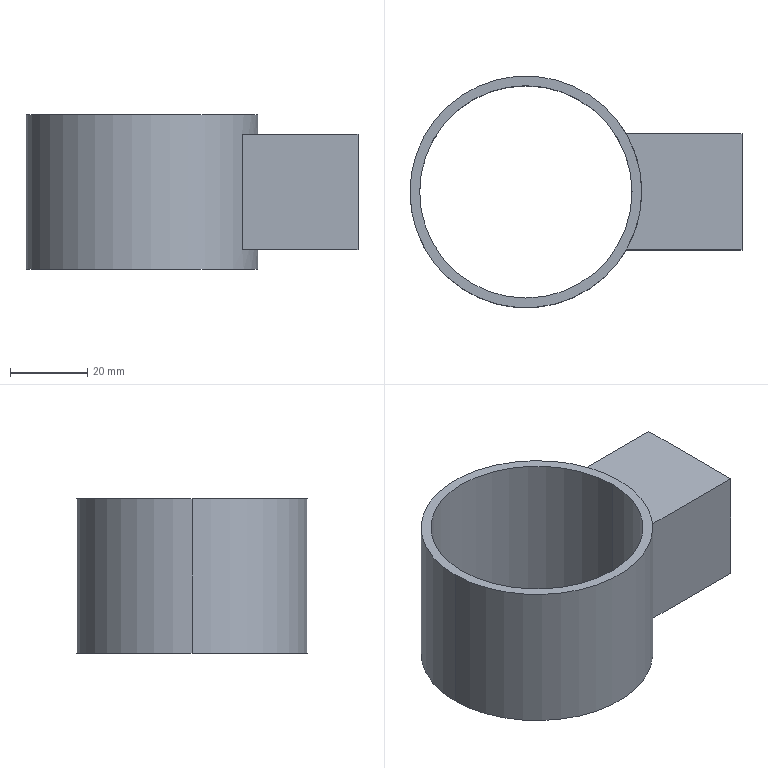Component | SolidWorks | 7TutorialFrame-1 | 1 solid | 16 faces | box 85.98 x 60 x 40 mm | volume 24052 mm3 | plane 11 | cylinder 5 | commonest cylinder face diameters 55 x2 60 x2 59 x1
STEP:
#1=CARTESIAN_POINT('',(4.528,-32.334,23.728));
#2=VERTEX_POINT('',#1);
#3=CARTESIAN_POINT('',(6.693,-32.334,23.728));
#4=VERTEX_POINT('',#3);
#5=CARTESIAN_POINT('',(5.61,-32.334,23.728));
#6=DIRECTION('',(0.,0.,1.));
#7=DIRECTION('',(1.,0.,0.));
#8=AXIS2_PLACEMENT_3D('',#5,#6,#7);
#9=CIRCLE('',#8,1.083);
#10=EDGE_CURVE('',#2,#4,#9,.T.);
#11=ORIENTED_EDGE('',*,*,#10,.T.);
#12=CARTESIAN_POINT('',(6.693,-32.334,22.153));
#13=VERTEX_POINT('',#12);
#14=CARTESIAN_POINT('',(6.693,-32.334,23.728));
#15=DIRECTION('',(0.,0.,-1.));
#16=VECTOR('',#15,39.37);
#17=LINE('',#14,#16);
#18=EDGE_CURVE('',#4,#13,#17,.T.);
#19=ORIENTED_EDGE('',*,*,#18,.T.);
#20=CARTESIAN_POINT('',(4.528,-32.334,22.153));
#21=VERTEX_POINT('',#20);
#22=CARTESIAN_POINT('',(5.61,-32.334,22.153));
#23=DIRECTION('',(0.,0.,1.));
#24=DIRECTION('',(1.,0.,0.));
#25=AXIS2_PLACEMENT_3D('',#22,#23,#24);
#26=CIRCLE('',#25,1.083);
#27=EDGE_CURVE('',#21,#13,#26,.T.);
#28=ORIENTED_EDGE('',*,*,#27,.F.);
#29=CARTESIAN_POINT('',(4.528,-32.334,23.728));
#30=DIRECTION('',(0.,0.,-1.));
#31=VECTOR('',#30,39.37);
#32=LINE('',#29,#31);
#33=EDGE_CURVE('',#2,#21,#32,.T.);
#34=ORIENTED_EDGE('',*,*,#33,.F.);
#35=EDGE_LOOP('',(#11,#19,#28,#34));
#36=FACE_OUTER_BOUND('',#35,.T.);
#37=CARTESIAN_POINT('',(5.61,-32.334,23.728));
#38=DIRECTION('',(0.,0.,-1.));
#39=DIRECTION('',(-1.,0.,0.));
#40=AXIS2_PLACEMENT_3D('',#37,#38,#39);
#41=CYLINDRICAL_SURFACE('',#40,1.083);
#42=ADVANCED_FACE('',(#36),#41,.F.);
#43=CARTESIAN_POINT('',(6.791,-32.334,23.728));
#44=VERTEX_POINT('',#43);
#45=CARTESIAN_POINT('',(4.429,-32.334,23.728));
#46=VERTEX_POINT('',#45);
#47=CARTESIAN_POINT('',(5.61,-32.334,23.728));
#48=DIRECTION('',(0.,0.,1.));
#49=DIRECTION('',(1.,0.,0.));
#50=AXIS2_PLACEMENT_3D('',#47,#48,#49);
#51=CIRCLE('',#50,1.181);
#52=EDGE_CURVE('',#44,#46,#51,.T.);
#53=ORIENTED_EDGE('',*,*,#52,.F.);
#54=CARTESIAN_POINT('',(6.791,-32.334,23.531));
#55=VERTEX_POINT('',#54);
#56=CARTESIAN_POINT('',(6.791,-32.334,23.728));
#57=DIRECTION('',(0.,0.,-1.));
#58=VECTOR('',#57,39.37);
#59=LINE('',#56,#58);
#60=EDGE_CURVE('',#44,#55,#59,.T.);
#61=ORIENTED_EDGE('',*,*,#60,.T.);
#62=CARTESIAN_POINT('',(6.633,-31.744,23.531));
#63=VERTEX_POINT('',#62);
#64=CARTESIAN_POINT('',(5.61,-32.334,23.531));
#65=DIRECTION('',(0.,0.,1.));
#66=DIRECTION('',(1.,0.,0.));
#67=AXIS2_PLACEMENT_3D('',#64,#65,#66);
#68=CIRCLE('',#67,1.181);
#69=EDGE_CURVE('',#55,#63,#68,.T.);
#70=ORIENTED_EDGE('',*,*,#69,.T.);
#71=CARTESIAN_POINT('',(6.633,-31.744,22.35));
#72=VERTEX_POINT('',#71);
#73=CARTESIAN_POINT('',(6.633,-31.744,23.531));
#74=DIRECTION('',(0.,0.,-1.));
#75=VECTOR('',#74,39.37);
#76=LINE('',#73,#75);
#77=EDGE_CURVE('',#63,#72,#76,.T.);
#78=ORIENTED_EDGE('',*,*,#77,.T.);
#79=CARTESIAN_POINT('',(6.791,-32.334,22.35));
#80=VERTEX_POINT('',#79);
#81=CARTESIAN_POINT('',(5.61,-32.334,22.35));
#82=DIRECTION('',(0.,0.,1.));
#83=DIRECTION('',(1.,0.,0.));
#84=AXIS2_PLACEMENT_3D('',#81,#82,#83);
#85=CIRCLE('',#84,1.181);
#86=EDGE_CURVE('',#80,#72,#85,.T.);
#87=ORIENTED_EDGE('',*,*,#86,.F.);
#88=CARTESIAN_POINT('',(6.791,-32.334,22.153));
#89=VERTEX_POINT('',#88);
#90=CARTESIAN_POINT('',(6.791,-32.334,23.728));
#91=DIRECTION('',(0.,0.,-1.));
#92=VECTOR('',#91,39.37);
#93=LINE('',#90,#92);
#94=EDGE_CURVE('',#80,#89,#93,.T.);
#95=ORIENTED_EDGE('',*,*,#94,.T.);
#96=CARTESIAN_POINT('',(4.429,-32.334,22.153));
#97=VERTEX_POINT('',#96);
#98=CARTESIAN_POINT('',(5.61,-32.334,22.153));
#99=DIRECTION('',(0.,0.,1.));
#100=DIRECTION('',(1.,0.,0.));
#101=AXIS2_PLACEMENT_3D('',#98,#99,#100);
#102=CIRCLE('',#101,1.181);
#103=EDGE_CURVE('',#89,#97,#102,.T.);
#104=ORIENTED_EDGE('',*,*,#103,.T.);
#105=CARTESIAN_POINT('',(4.429,-32.334,23.728));
#106=DIRECTION('',(0.,0.,-1.));
#107=VECTOR('',#106,39.37);
#108=LINE('',#105,#107);
#109=EDGE_CURVE('',#46,#97,#108,.T.);
#110=ORIENTED_EDGE('',*,*,#109,.F.);
#111=EDGE_LOOP('',(#53,#61,#70,#78,#87,#95,#104,#110));
#112=FACE_OUTER_BOUND('',#111,.T.);
#113=CARTESIAN_POINT('',(5.61,-32.334,23.728));
#114=DIRECTION('',(0.,0.,-1.));
#115=DIRECTION('',(-1.,0.,0.));
#116=AXIS2_PLACEMENT_3D('',#113,#114,#115);
#117=CYLINDRICAL_SURFACE('',#116,1.181);
#118=ADVANCED_FACE('',(#112),#117,.T.);
#119=CARTESIAN_POINT('',(7.814,-31.744,22.35));
#120=VERTEX_POINT('',#119);
#121=CARTESIAN_POINT('',(7.814,-32.925,22.35));
#122=VERTEX_POINT('',#121);
#123=CARTESIAN_POINT('',(7.814,-32.334,22.35));
#124=DIRECTION('',(0.,-1.,0.));
#125=VECTOR('',#124,39.37);
#126=LINE('',#123,#125);
#127=EDGE_CURVE('',#120,#122,#126,.T.);
#128=ORIENTED_EDGE('',*,*,#127,.F.);
#129=CARTESIAN_POINT('',(7.814,-31.744,23.531));
#130=VERTEX_POINT('',#129);
#131=CARTESIAN_POINT('',(7.814,-31.744,23.531));
#132=DIRECTION('',(0.,0.,-1.));
#133=VECTOR('',#132,39.37);
#134=LINE('',#131,#133);
#135=EDGE_CURVE('',#130,#120,#134,.T.);
#136=ORIENTED_EDGE('',*,*,#135,.F.);
#137=CARTESIAN_POINT('',(7.814,-32.925,23.531));
#138=VERTEX_POINT('',#137);
#139=CARTESIAN_POINT('',(7.814,-32.334,23.531));
#140=DIRECTION('',(0.,-1.,0.));
#141=VECTOR('',#140,39.37);
#142=LINE('',#139,#141);
#143=EDGE_CURVE('',#130,#138,#142,.T.);
#144=ORIENTED_EDGE('',*,*,#143,.T.);
#145=CARTESIAN_POINT('',(7.814,-32.925,23.531));
#146=DIRECTION('',(0.,0.,-1.));
#147=VECTOR('',#146,39.37);
#148=LINE('',#145,#147);
#149=EDGE_CURVE('',#138,#122,#148,.T.);
#150=ORIENTED_EDGE('',*,*,#149,.T.);
#151=EDGE_LOOP('',(#128,#136,#144,#150));
#152=FACE_OUTER_BOUND('',#151,.T.);
#153=CARTESIAN_POINT('',(7.814,-31.822,23.452));
#154=VERTEX_POINT('',#153);
#155=CARTESIAN_POINT('',(7.814,-31.822,22.428));
#156=VERTEX_POINT('',#155);
#157=CARTESIAN_POINT('',(7.814,-31.822,23.531));
#158=DIRECTION('',(0.,0.,-1.));
#159=VECTOR('',#158,39.37);
#160=LINE('',#157,#159);
#161=EDGE_CURVE('',#154,#156,#160,.T.);
#162=ORIENTED_EDGE('',*,*,#161,.T.);
#163=CARTESIAN_POINT('',(7.814,-32.846,22.428));
#164=VERTEX_POINT('',#163);
#165=CARTESIAN_POINT('',(7.814,-32.334,22.428));
#166=DIRECTION('',(0.,-1.,0.));
#167=VECTOR('',#166,39.37);
#168=LINE('',#165,#167);
#169=EDGE_CURVE('',#156,#164,#168,.T.);
#170=ORIENTED_EDGE('',*,*,#169,.T.);
#171=CARTESIAN_POINT('',(7.814,-32.846,23.452));
#172=VERTEX_POINT('',#171);
#173=CARTESIAN_POINT('',(7.814,-32.846,23.531));
#174=DIRECTION('',(0.,0.,-1.));
#175=VECTOR('',#174,39.37);
#176=LINE('',#173,#175);
#177=EDGE_CURVE('',#172,#164,#176,.T.);
#178=ORIENTED_EDGE('',*,*,#177,.F.);
#179=CARTESIAN_POINT('',(7.814,-32.334,23.452));
#180=DIRECTION('',(0.,-1.,0.));
#181=VECTOR('',#180,39.37);
#182=LINE('',#179,#181);
#183=EDGE_CURVE('',#154,#172,#182,.T.);
#184=ORIENTED_EDGE('',*,*,#183,.F.);
#185=EDGE_LOOP('',(#162,#170,#178,#184));
#186=FACE_BOUND('',#185,.T.);
#187=CARTESIAN_POINT('',(7.814,-32.334,23.531));
#188=DIRECTION('',(1.,0.,0.));
#189=DIRECTION('',(0.,0.,-1.));
#190=AXIS2_PLACEMENT_3D('',#187,#188,#189);
#191=PLANE('',#190);
#192=ADVANCED_FACE('',(#152,#186),#191,.T.);
#193=ORIENTED_EDGE('',*,*,#60,.F.);
#194=CARTESIAN_POINT('',(5.61,-32.334,23.728));
#195=DIRECTION('',(0.,0.,1.));
#196=DIRECTION('',(1.,0.,0.));
#197=AXIS2_PLACEMENT_3D('',#194,#195,#196);
#198=CIRCLE('',#197,1.181);
#199=EDGE_CURVE('',#46,#44,#198,.T.);
#200=ORIENTED_EDGE('',*,*,#199,.F.);
#201=ORIENTED_EDGE('',*,*,#109,.T.);
#202=CARTESIAN_POINT('',(5.61,-32.334,22.153));
#203=DIRECTION('',(0.,0.,1.));
#204=DIRECTION('',(1.,0.,0.));
#205=AXIS2_PLACEMENT_3D('',#202,#203,#204);
#206=CIRCLE('',#205,1.181);
#207=EDGE_CURVE('',#97,#89,#206,.T.);
#208=ORIENTED_EDGE('',*,*,#207,.T.);
#209=ORIENTED_EDGE('',*,*,#94,.F.);
#210=CARTESIAN_POINT('',(6.633,-32.925,22.35));
#211=VERTEX_POINT('',#210);
#212=CARTESIAN_POINT('',(5.61,-32.334,22.35));
#213=DIRECTION('',(0.,0.,1.));
#214=DIRECTION('',(1.,0.,0.));
#215=AXIS2_PLACEMENT_3D('',#212,#213,#214);
#216=CIRCLE('',#215,1.181);
#217=EDGE_CURVE('',#211,#80,#216,.T.);
#218=ORIENTED_EDGE('',*,*,#217,.F.);
#219=CARTESIAN_POINT('',(6.633,-32.925,23.531));
#220=VERTEX_POINT('',#219);
#221=CARTESIAN_POINT('',(6.633,-32.925,23.531));
#222=DIRECTION('',(0.,0.,-1.));
#223=VECTOR('',#222,39.37);
#224=LINE('',#221,#223);
#225=EDGE_CURVE('',#220,#211,#224,.T.);
#226=ORIENTED_EDGE('',*,*,#225,.F.);
#227=CARTESIAN_POINT('',(5.61,-32.334,23.531));
#228=DIRECTION('',(0.,0.,1.));
#229=DIRECTION('',(1.,0.,0.));
#230=AXIS2_PLACEMENT_3D('',#227,#228,#229);
#231=CIRCLE('',#230,1.181);
#232=EDGE_CURVE('',#220,#55,#231,.T.);
#233=ORIENTED_EDGE('',*,*,#232,.T.);
#234=EDGE_LOOP('',(#193,#200,#201,#208,#209,#218,#226,#233));
#235=FACE_OUTER_BOUND('',#234,.T.);
#236=CARTESIAN_POINT('',(5.61,-32.334,23.728));
#237=DIRECTION('',(0.,0.,-1.));
#238=DIRECTION('',(-1.,0.,0.));
#239=AXIS2_PLACEMENT_3D('',#236,#237,#238);
#240=CYLINDRICAL_SURFACE('',#239,1.181);
#241=ADVANCED_FACE('',(#235),#240,.T.);
#242=ORIENTED_EDGE('',*,*,#18,.F.);
#243=CARTESIAN_POINT('',(5.61,-32.334,23.728));
#244=DIRECTION('',(0.,0.,1.));
#245=DIRECTION('',(1.,0.,0.));
#246=AXIS2_PLACEMENT_3D('',#243,#244,#245);
#247=CIRCLE('',#246,1.083);
#248=EDGE_CURVE('',#4,#2,#247,.T.);
#249=ORIENTED_EDGE('',*,*,#248,.T.);
#250=ORIENTED_EDGE('',*,*,#33,.T.);
#251=CARTESIAN_POINT('',(5.61,-32.334,22.153));
#252=DIRECTION('',(0.,0.,1.));
#253=DIRECTION('',(1.,0.,0.));
#254=AXIS2_PLACEMENT_3D('',#251,#252,#253);
#255=CIRCLE('',#254,1.083);
#256=EDGE_CURVE('',#13,#21,#255,.T.);
#257=ORIENTED_EDGE('',*,*,#256,.F.);
#258=EDGE_LOOP('',(#242,#249,#250,#257));
#259=FACE_OUTER_BOUND('',#258,.T.);
#260=CARTESIAN_POINT('',(5.61,-32.334,23.728));
#261=DIRECTION('',(0.,0.,-1.));
#262=DIRECTION('',(-1.,0.,0.));
#263=AXIS2_PLACEMENT_3D('',#260,#261,#262);
#264=CYLINDRICAL_SURFACE('',#263,1.083);
#265=ADVANCED_FACE('',(#259),#264,.F.);
#266=ORIENTED_EDGE('',*,*,#199,.T.);
#267=ORIENTED_EDGE('',*,*,#52,.T.);
#268=EDGE_LOOP('',(#266,#267));
#269=FACE_OUTER_BOUND('',#268,.T.);
#270=ORIENTED_EDGE('',*,*,#10,.F.);
#271=ORIENTED_EDGE('',*,*,#248,.F.);
#272=EDGE_LOOP('',(#270,#271));
#273=FACE_BOUND('',#272,.T.);
#274=CARTESIAN_POINT('',(5.61,-32.334,23.728));
#275=DIRECTION('',(0.,0.,1.));
#276=DIRECTION('',(1.,0.,0.));
#277=AXIS2_PLACEMENT_3D('',#274,#275,#276);
#278=PLANE('',#277);
#279=ADVANCED_FACE('',(#269,#273),#278,.T.);
#280=ORIENTED_EDGE('',*,*,#207,.F.);
#281=ORIENTED_EDGE('',*,*,#103,.F.);
#282=EDGE_LOOP('',(#280,#281));
#283=FACE_OUTER_BOUND('',#282,.T.);
#284=ORIENTED_EDGE('',*,*,#27,.T.);
#285=ORIENTED_EDGE('',*,*,#256,.T.);
#286=EDGE_LOOP('',(#284,#285));
#287=FACE_BOUND('',#286,.T.);
#288=CARTESIAN_POINT('',(5.61,-32.334,22.153));
#289=DIRECTION('',(0.,0.,1.));
#290=DIRECTION('',(1.,0.,0.));
#291=AXIS2_PLACEMENT_3D('',#288,#289,#290);
#292=PLANE('',#291);
#293=ADVANCED_FACE('',(#283,#287),#292,.F.);
#294=CARTESIAN_POINT('',(5.61,-31.744,22.35));
#295=DIRECTION('',(1.,0.,0.));
#296=VECTOR('',#295,39.37);
#297=LINE('',#294,#296);
#298=EDGE_CURVE('',#72,#120,#297,.T.);
#299=ORIENTED_EDGE('',*,*,#298,.F.);
#300=ORIENTED_EDGE('',*,*,#77,.F.);
#301=CARTESIAN_POINT('',(5.61,-31.744,23.531));
#302=DIRECTION('',(1.,0.,0.));
#303=VECTOR('',#302,39.37);
#304=LINE('',#301,#303);
#305=EDGE_CURVE('',#63,#130,#304,.T.);
#306=ORIENTED_EDGE('',*,*,#305,.T.);
#307=ORIENTED_EDGE('',*,*,#135,.T.);
#308=EDGE_LOOP('',(#299,#300,#306,#307));
#309=FACE_OUTER_BOUND('',#308,.T.);
#310=CARTESIAN_POINT('',(5.61,-31.744,23.531));
#311=DIRECTION('',(-0.,1.,0.));
#312=DIRECTION('',(-1.,-0.,0.));
#313=AXIS2_PLACEMENT_3D('',#310,#311,#312);
#314=PLANE('',#313);
#315=ADVANCED_FACE('',(#309),#314,.T.);
#316=CARTESIAN_POINT('',(5.61,-32.925,22.35));
#317=DIRECTION('',(1.,-0.,0.));
#318=VECTOR('',#317,39.37);
#319=LINE('',#316,#318);
#320=EDGE_CURVE('',#211,#122,#319,.T.);
#321=ORIENTED_EDGE('',*,*,#320,.T.);
#322=ORIENTED_EDGE('',*,*,#149,.F.);
#323=CARTESIAN_POINT('',(5.61,-32.925,23.531));
#324=DIRECTION('',(1.,-0.,0.));
#325=VECTOR('',#324,39.37);
#326=LINE('',#323,#325);
#327=EDGE_CURVE('',#220,#138,#326,.T.);
#328=ORIENTED_EDGE('',*,*,#327,.F.);
#329=ORIENTED_EDGE('',*,*,#225,.T.);
#330=EDGE_LOOP('',(#321,#322,#328,#329));
#331=FACE_OUTER_BOUND('',#330,.T.);
#332=CARTESIAN_POINT('',(5.61,-32.925,23.531));
#333=DIRECTION('',(0.,1.,0.));
#334=DIRECTION('',(-1.,0.,0.));
#335=AXIS2_PLACEMENT_3D('',#332,#333,#334);
#336=PLANE('',#335);
#337=ADVANCED_FACE('',(#331),#336,.F.);
#338=ORIENTED_EDGE('',*,*,#143,.F.);
#339=ORIENTED_EDGE('',*,*,#305,.F.);
#340=ORIENTED_EDGE('',*,*,#69,.F.);
#341=ORIENTED_EDGE('',*,*,#232,.F.);
#342=ORIENTED_EDGE('',*,*,#327,.T.);
#343=EDGE_LOOP('',(#338,#339,#340,#341,#342));
#344=FACE_OUTER_BOUND('',#343,.T.);
#345=CARTESIAN_POINT('',(5.61,-32.334,23.531));
#346=DIRECTION('',(0.,0.,1.));
#347=DIRECTION('',(1.,0.,0.));
#348=AXIS2_PLACEMENT_3D('',#345,#346,#347);
#349=PLANE('',#348);
#350=ADVANCED_FACE('',(#344),#349,.T.);
#351=ORIENTED_EDGE('',*,*,#127,.T.);
#352=ORIENTED_EDGE('',*,*,#320,.F.);
#353=ORIENTED_EDGE('',*,*,#217,.T.);
#354=ORIENTED_EDGE('',*,*,#86,.T.);
#355=ORIENTED_EDGE('',*,*,#298,.T.);
#356=EDGE_LOOP('',(#351,#352,#353,#354,#355));
#357=FACE_OUTER_BOUND('',#356,.T.);
#358=CARTESIAN_POINT('',(5.61,-32.334,22.35));
#359=DIRECTION('',(0.,0.,1.));
#360=DIRECTION('',(1.,0.,0.));
#361=AXIS2_PLACEMENT_3D('',#358,#359,#360);
#362=PLANE('',#361);
#363=ADVANCED_FACE('',(#357),#362,.F.);
#364=CARTESIAN_POINT('',(6.653,-32.846,22.428));
#365=VERTEX_POINT('',#364);
#366=CARTESIAN_POINT('',(5.61,-32.846,22.428));
#367=DIRECTION('',(1.,-0.,0.));
#368=VECTOR('',#367,39.37);
#369=LINE('',#366,#368);
#370=EDGE_CURVE('',#365,#164,#369,.T.);
#371=ORIENTED_EDGE('',*,*,#370,.T.);
#372=ORIENTED_EDGE('',*,*,#169,.F.);
#373=CARTESIAN_POINT('',(6.653,-31.822,22.428));
#374=VERTEX_POINT('',#373);
#375=CARTESIAN_POINT('',(5.61,-31.822,22.428));
#376=DIRECTION('',(1.,0.,0.));
#377=VECTOR('',#376,39.37);
#378=LINE('',#375,#377);
#379=EDGE_CURVE('',#374,#156,#378,.T.);
#380=ORIENTED_EDGE('',*,*,#379,.F.);
#381=CARTESIAN_POINT('',(5.61,-32.334,22.428));
#382=DIRECTION('',(0.,0.,1.));
#383=DIRECTION('',(1.,0.,0.));
#384=AXIS2_PLACEMENT_3D('',#381,#382,#383);
#385=CIRCLE('',#384,1.161);
#386=EDGE_CURVE('',#365,#374,#385,.T.);
#387=ORIENTED_EDGE('',*,*,#386,.F.);
#388=EDGE_LOOP('',(#371,#372,#380,#387));
#389=FACE_OUTER_BOUND('',#388,.T.);
#390=CARTESIAN_POINT('',(5.61,-32.334,22.428));
#391=DIRECTION('',(0.,0.,1.));
#392=DIRECTION('',(1.,0.,0.));
#393=AXIS2_PLACEMENT_3D('',#390,#391,#392);
#394=PLANE('',#393);
#395=ADVANCED_FACE('',(#389),#394,.T.);
#396=CARTESIAN_POINT('',(6.653,-31.822,23.452));
#397=VERTEX_POINT('',#396);
#398=CARTESIAN_POINT('',(6.653,-31.822,23.728));
#399=DIRECTION('',(0.,0.,-1.));
#400=VECTOR('',#399,39.37);
#401=LINE('',#398,#400);
#402=EDGE_CURVE('',#397,#374,#401,.T.);
#403=ORIENTED_EDGE('',*,*,#402,.T.);
#404=ORIENTED_EDGE('',*,*,#379,.T.);
#405=ORIENTED_EDGE('',*,*,#161,.F.);
#406=CARTESIAN_POINT('',(5.61,-31.822,23.452));
#407=DIRECTION('',(1.,0.,0.));
#408=VECTOR('',#407,39.37);
#409=LINE('',#406,#408);
#410=EDGE_CURVE('',#397,#154,#409,.T.);
#411=ORIENTED_EDGE('',*,*,#410,.F.);
#412=EDGE_LOOP('',(#403,#404,#405,#411));
#413=FACE_OUTER_BOUND('',#412,.T.);
#414=CARTESIAN_POINT('',(5.61,-31.822,23.531));
#415=DIRECTION('',(-0.,1.,0.));
#416=DIRECTION('',(-1.,-0.,0.));
#417=AXIS2_PLACEMENT_3D('',#414,#415,#416);
#418=PLANE('',#417);
#419=ADVANCED_FACE('',(#413),#418,.F.);
#420=CARTESIAN_POINT('',(6.653,-32.846,23.452));
#421=VERTEX_POINT('',#420);
#422=CARTESIAN_POINT('',(5.61,-32.334,23.452));
#423=DIRECTION('',(0.,0.,1.));
#424=DIRECTION('',(1.,0.,0.));
#425=AXIS2_PLACEMENT_3D('',#422,#423,#424);
#426=CIRCLE('',#425,1.161);
#427=EDGE_CURVE('',#421,#397,#426,.T.);
#428=ORIENTED_EDGE('',*,*,#427,.T.);
#429=ORIENTED_EDGE('',*,*,#410,.T.);
#430=ORIENTED_EDGE('',*,*,#183,.T.);
#431=CARTESIAN_POINT('',(5.61,-32.846,23.452));
#432=DIRECTION('',(1.,-0.,0.));
#433=VECTOR('',#432,39.37);
#434=LINE('',#431,#433);
#435=EDGE_CURVE('',#421,#172,#434,.T.);
#436=ORIENTED_EDGE('',*,*,#435,.F.);
#437=EDGE_LOOP('',(#428,#429,#430,#436));
#438=FACE_OUTER_BOUND('',#437,.T.);
#439=CARTESIAN_POINT('',(5.61,-32.334,23.452));
#440=DIRECTION('',(0.,0.,1.));
#441=DIRECTION('',(1.,0.,0.));
#442=AXIS2_PLACEMENT_3D('',#439,#440,#441);
#443=PLANE('',#442);
#444=ADVANCED_FACE('',(#438),#443,.F.);
#445=ORIENTED_EDGE('',*,*,#435,.T.);
#446=ORIENTED_EDGE('',*,*,#177,.T.);
#447=ORIENTED_EDGE('',*,*,#370,.F.);
#448=CARTESIAN_POINT('',(6.653,-32.846,23.728));
#449=DIRECTION('',(0.,0.,-1.));
#450=VECTOR('',#449,39.37);
#451=LINE('',#448,#450);
#452=EDGE_CURVE('',#421,#365,#451,.T.);
#453=ORIENTED_EDGE('',*,*,#452,.F.);
#454=EDGE_LOOP('',(#445,#446,#447,#453));
#455=FACE_OUTER_BOUND('',#454,.T.);
#456=CARTESIAN_POINT('',(5.61,-32.846,23.531));
#457=DIRECTION('',(0.,1.,0.));
#458=DIRECTION('',(-1.,0.,0.));
#459=AXIS2_PLACEMENT_3D('',#456,#457,#458);
#460=PLANE('',#459);
#461=ADVANCED_FACE('',(#455),#460,.T.);
#462=ORIENTED_EDGE('',*,*,#386,.T.);
#463=ORIENTED_EDGE('',*,*,#402,.F.);
#464=ORIENTED_EDGE('',*,*,#427,.F.);
#465=ORIENTED_EDGE('',*,*,#452,.T.);
#466=EDGE_LOOP('',(#462,#463,#464,#465));
#467=FACE_OUTER_BOUND('',#466,.T.);
#468=CARTESIAN_POINT('',(5.61,-32.334,23.728));
#469=DIRECTION('',(0.,0.,-1.));
#470=DIRECTION('',(-1.,0.,0.));
#471=AXIS2_PLACEMENT_3D('',#468,#469,#470);
#472=CYLINDRICAL_SURFACE('',#471,1.161);
#473=ADVANCED_FACE('',(#467),#472,.T.);
#474=CLOSED_SHELL('',(#42,#118,#192,#241,#265,#279,#293,#315,#337,#350,#363,#395,#419,#444,#461,#473));
#475=MANIFOLD_SOLID_BREP('',#474);
#476=CARTESIAN_POINT('',(0.,0.,0.));
#477=DIRECTION('',(0.,0.,1.));
#478=DIRECTION('',(1.,0.,0.));
#479=AXIS2_PLACEMENT_3D('',#476,#477,#478);
#480=(LENGTH_UNIT()NAMED_UNIT(*)SI_UNIT($,.METRE.));
#481=LENGTH_MEASURE_WITH_UNIT(LENGTH_MEASURE(0.0254),#480);
#482=DIMENSIONAL_EXPONENTS(1.,0.,0.,0.,0.,0.,0.);
#483=(CONVERSION_BASED_UNIT('',#481)LENGTH_UNIT()NAMED_UNIT(#482));
#484=UNCERTAINTY_MEASURE_WITH_UNIT(LENGTH_MEASURE(0.00001),#483,'','');
#485=(NAMED_UNIT(*)PLANE_ANGLE_UNIT()SI_UNIT($,.RADIAN.));
#486=(NAMED_UNIT(*)SI_UNIT($,.STERADIAN.)SOLID_ANGLE_UNIT());
#487=(GEOMETRIC_REPRESENTATION_CONTEXT(3)GLOBAL_UNCERTAINTY_ASSIGNED_CONTEXT((#484))GLOBAL_UNIT_ASSIGNED_CONTEXT((#483,#485,#486))REPRESENTATION_CONTEXT('',''));
#488=ADVANCED_BREP_SHAPE_REPRESENTATION('',(#475,#479),#487);
#489=COLOUR_RGB('',0.7922,0.8196,0.9333);
#490=FILL_AREA_STYLE_COLOUR('',#489);
#491=FILL_AREA_STYLE('',(#490));
#492=SURFACE_STYLE_FILL_AREA(#491);
#493=SURFACE_SIDE_STYLE('',(#492));
#494=SURFACE_STYLE_USAGE(.BOTH.,#493);
#495=PRESENTATION_STYLE_ASSIGNMENT((#494));
#496=STYLED_ITEM('',(#495),#475);
#497=(LENGTH_UNIT()NAMED_UNIT(*)SI_UNIT($,.METRE.));
#498=LENGTH_MEASURE_WITH_UNIT(LENGTH_MEASURE(0.0254),#497);
#499=DIMENSIONAL_EXPONENTS(1.,0.,0.,0.,0.,0.,0.);
#500=(CONVERSION_BASED_UNIT('',#498)LENGTH_UNIT()NAMED_UNIT(#499));
#501=UNCERTAINTY_MEASURE_WITH_UNIT(LENGTH_MEASURE(0.00001),#500,'','');
#502=(NAMED_UNIT(*)PLANE_ANGLE_UNIT()SI_UNIT($,.RADIAN.));
#503=(NAMED_UNIT(*)SI_UNIT($,.STERADIAN.)SOLID_ANGLE_UNIT());
#504=(GEOMETRIC_REPRESENTATION_CONTEXT(3)GLOBAL_UNCERTAINTY_ASSIGNED_CONTEXT((#501))GLOBAL_UNIT_ASSIGNED_CONTEXT((#500,#502,#503))REPRESENTATION_CONTEXT('',''));
#505=MECHANICAL_DESIGN_GEOMETRIC_PRESENTATION_REPRESENTATION('',(#496),#504);
#506=PRESENTATION_LAYER_ASSIGNMENT('','',(#496));